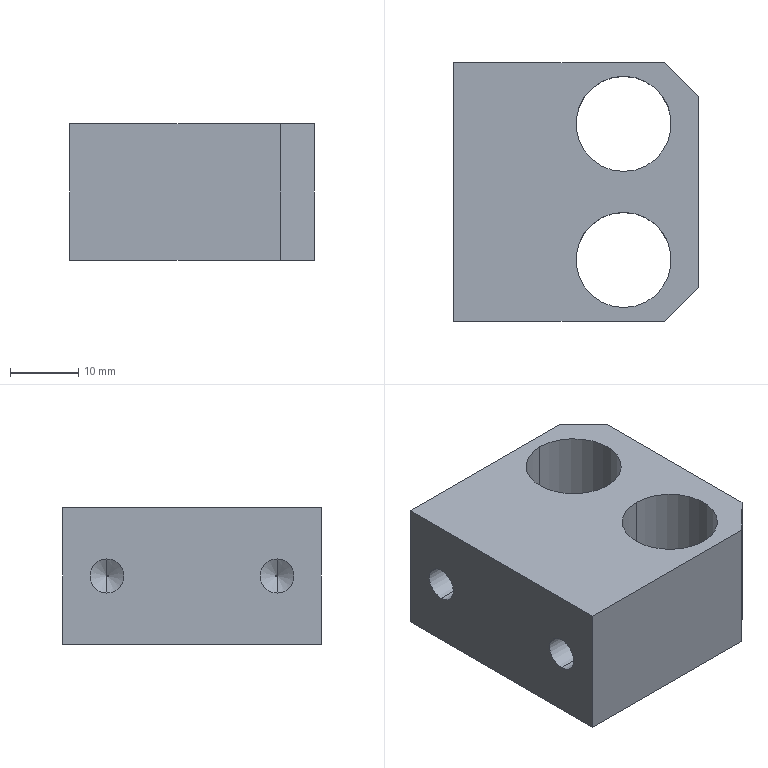Component | SolidWorks | 51-1 | 1 solid | 20 faces | box 36 x 38 x 20 mm | volume 20015 mm3 | cylinder 8 | plane 8 | cone 4 | commonest cylinder face diameters 14 x4 5 x4
build123d program:
from build123d import *

# Parameters (mm, degrees)
SKETCH1_W             = 38
SKETCH1_H             = 36
BOSS_EXTRUDE1_DEPTH   = 20
M6_TAPPED_HOLE1_D     = 5
M6_TAPPED_HOLE1_DEPTH = 17
M6_TAPPED_HOLE1_TIP   = 1.502
SKETCH4_R             = 7
CUT_EXTRUDE1_DEPTH    = 20
CHAMFER1_SIZE         = 5


with BuildPart() as part:
    # Sketch1 → Boss-Extrude1 (new body)
    with BuildSketch(Plane.XY):
        Rectangle(SKETCH1_W, SKETCH1_H)
    extrude(amount=BOSS_EXTRUDE1_DEPTH)

    # M6 Tapped Hole1
    with Locations(Plane(origin=(0, 18, 0), x_dir=(1, 0, 0), z_dir=(0, 1, 0))):
        with Locations((-12.5, -10), (12.5, -10)):
            Hole(M6_TAPPED_HOLE1_D / 2, depth=M6_TAPPED_HOLE1_DEPTH)
            with Locations((0, 0, -(M6_TAPPED_HOLE1_DEPTH + M6_TAPPED_HOLE1_TIP / 2))):  # 118° drill point
                Cone(0, M6_TAPPED_HOLE1_D / 2, M6_TAPPED_HOLE1_TIP, mode=Mode.SUBTRACT)

    # Sketch4 → Cut-Extrude1 (cut)
    with BuildSketch(Plane.XY.offset(20)):
        with Locations((-10, -7)):
            Circle(SKETCH4_R)
        with Locations((10, -7)):
            Circle(SKETCH4_R)
    extrude(amount=-CUT_EXTRUDE1_DEPTH, mode=Mode.SUBTRACT)

    # Chamfer1
    chamfer1_edges = [part.edges().sort_by_distance(p)[0] for p in [
        (19, -18, 10),
        (-19, -18, 10),
    ]]
    chamfer(chamfer1_edges, length=CHAMFER1_SIZE)


solid = part.part

# Placed as in the assembly
solid = solid.moved(Location((-7, -28, 376.398), (0, 0, 90)))
STEP:
#1=CARTESIAN_POINT('',(-0.,-0.9843,14.819));
#2=VERTEX_POINT('',#1);
#3=CARTESIAN_POINT('',(0.,-0.4331,14.819));
#4=VERTEX_POINT('',#3);
#5=CARTESIAN_POINT('',(-0.,-0.7087,14.819));
#6=DIRECTION('',(0.,0.,1.));
#7=DIRECTION('',(0.,1.,0.));
#8=AXIS2_PLACEMENT_3D('',#5,#6,#7);
#9=CIRCLE('',#8,0.2756);
#10=EDGE_CURVE('',#2,#4,#9,.T.);
#11=ORIENTED_EDGE('',*,*,#10,.F.);
#12=CARTESIAN_POINT('',(-0.,-0.9843,15.606));
#13=VERTEX_POINT('',#12);
#14=CARTESIAN_POINT('',(-0.,-0.9843,14.819));
#15=DIRECTION('',(0.,0.,1.));
#16=VECTOR('',#15,39.37);
#17=LINE('',#14,#16);
#18=EDGE_CURVE('',#2,#13,#17,.T.);
#19=ORIENTED_EDGE('',*,*,#18,.T.);
#20=CARTESIAN_POINT('',(0.,-0.4331,15.606));
#21=VERTEX_POINT('',#20);
#22=CARTESIAN_POINT('',(-0.,-0.7087,15.606));
#23=DIRECTION('',(0.,0.,1.));
#24=DIRECTION('',(0.,1.,0.));
#25=AXIS2_PLACEMENT_3D('',#22,#23,#24);
#26=CIRCLE('',#25,0.2756);
#27=EDGE_CURVE('',#13,#21,#26,.T.);
#28=ORIENTED_EDGE('',*,*,#27,.T.);
#29=CARTESIAN_POINT('',(0.,-0.4331,14.819));
#30=DIRECTION('',(0.,0.,1.));
#31=VECTOR('',#30,39.37);
#32=LINE('',#29,#31);
#33=EDGE_CURVE('',#4,#21,#32,.T.);
#34=ORIENTED_EDGE('',*,*,#33,.F.);
#35=EDGE_LOOP('',(#11,#19,#28,#34));
#36=FACE_OUTER_BOUND('',#35,.T.);
#37=CARTESIAN_POINT('',(-0.,-0.7087,14.819));
#38=DIRECTION('',(0.,0.,1.));
#39=DIRECTION('',(0.,1.,0.));
#40=AXIS2_PLACEMENT_3D('',#37,#38,#39);
#41=CYLINDRICAL_SURFACE('',#40,0.2756);
#42=ADVANCED_FACE('',(#36),#41,.F.);
#43=CARTESIAN_POINT('',(-0.,-1.772,14.819));
#44=VERTEX_POINT('',#43);
#45=CARTESIAN_POINT('',(-0.,-1.22,14.819));
#46=VERTEX_POINT('',#45);
#47=CARTESIAN_POINT('',(-0.,-1.496,14.819));
#48=DIRECTION('',(0.,0.,1.));
#49=DIRECTION('',(0.,1.,0.));
#50=AXIS2_PLACEMENT_3D('',#47,#48,#49);
#51=CIRCLE('',#50,0.2756);
#52=EDGE_CURVE('',#44,#46,#51,.T.);
#53=ORIENTED_EDGE('',*,*,#52,.F.);
#54=CARTESIAN_POINT('',(-0.,-1.772,15.606));
#55=VERTEX_POINT('',#54);
#56=CARTESIAN_POINT('',(-0.,-1.772,14.819));
#57=DIRECTION('',(0.,0.,1.));
#58=VECTOR('',#57,39.37);
#59=LINE('',#56,#58);
#60=EDGE_CURVE('',#44,#55,#59,.T.);
#61=ORIENTED_EDGE('',*,*,#60,.T.);
#62=CARTESIAN_POINT('',(-0.,-1.22,15.606));
#63=VERTEX_POINT('',#62);
#64=CARTESIAN_POINT('',(-0.,-1.496,15.606));
#65=DIRECTION('',(0.,0.,1.));
#66=DIRECTION('',(0.,1.,0.));
#67=AXIS2_PLACEMENT_3D('',#64,#65,#66);
#68=CIRCLE('',#67,0.2756);
#69=EDGE_CURVE('',#55,#63,#68,.T.);
#70=ORIENTED_EDGE('',*,*,#69,.T.);
#71=CARTESIAN_POINT('',(-0.,-1.22,14.819));
#72=DIRECTION('',(0.,0.,1.));
#73=VECTOR('',#72,39.37);
#74=LINE('',#71,#73);
#75=EDGE_CURVE('',#46,#63,#74,.T.);
#76=ORIENTED_EDGE('',*,*,#75,.F.);
#77=EDGE_LOOP('',(#53,#61,#70,#76));
#78=FACE_OUTER_BOUND('',#77,.T.);
#79=CARTESIAN_POINT('',(-0.,-1.496,14.819));
#80=DIRECTION('',(0.,0.,1.));
#81=DIRECTION('',(0.,1.,0.));
#82=AXIS2_PLACEMENT_3D('',#79,#80,#81);
#83=CYLINDRICAL_SURFACE('',#82,0.2756);
#84=ADVANCED_FACE('',(#78),#83,.F.);
#85=CARTESIAN_POINT('',(-0.315,-1.594,15.114));
#86=VERTEX_POINT('',#85);
#87=CARTESIAN_POINT('',(-0.315,-1.594,15.311));
#88=VERTEX_POINT('',#87);
#89=CARTESIAN_POINT('',(-0.315,-1.594,15.213));
#90=DIRECTION('',(-1.,0.,0.));
#91=DIRECTION('',(0.,0.,1.));
#92=AXIS2_PLACEMENT_3D('',#89,#90,#91);
#93=CIRCLE('',#92,0.09843);
#94=EDGE_CURVE('',#86,#88,#93,.T.);
#95=ORIENTED_EDGE('',*,*,#94,.F.);
#96=CARTESIAN_POINT('',(-0.9843,-1.594,15.114));
#97=VERTEX_POINT('',#96);
#98=CARTESIAN_POINT('',(-0.9843,-1.594,15.114));
#99=DIRECTION('',(-1.,0.,0.));
#100=VECTOR('',#99,39.37);
#101=LINE('',#98,#100);
#102=EDGE_CURVE('',#86,#97,#101,.T.);
#103=ORIENTED_EDGE('',*,*,#102,.T.);
#104=CARTESIAN_POINT('',(-0.9843,-1.594,15.311));
#105=VERTEX_POINT('',#104);
#106=CARTESIAN_POINT('',(-0.9843,-1.594,15.213));
#107=DIRECTION('',(-1.,0.,0.));
#108=DIRECTION('',(0.,0.,1.));
#109=AXIS2_PLACEMENT_3D('',#106,#107,#108);
#110=CIRCLE('',#109,0.09843);
#111=EDGE_CURVE('',#97,#105,#110,.T.);
#112=ORIENTED_EDGE('',*,*,#111,.T.);
#113=CARTESIAN_POINT('',(-0.9843,-1.594,15.311));
#114=DIRECTION('',(-1.,0.,0.));
#115=VECTOR('',#114,39.37);
#116=LINE('',#113,#115);
#117=EDGE_CURVE('',#88,#105,#116,.T.);
#118=ORIENTED_EDGE('',*,*,#117,.F.);
#119=EDGE_LOOP('',(#95,#103,#112,#118));
#120=FACE_OUTER_BOUND('',#119,.T.);
#121=CARTESIAN_POINT('',(-0.9843,-1.594,15.213));
#122=DIRECTION('',(-1.,0.,0.));
#123=DIRECTION('',(0.,0.,1.));
#124=AXIS2_PLACEMENT_3D('',#121,#122,#123);
#125=CYLINDRICAL_SURFACE('',#124,0.09843);
#126=ADVANCED_FACE('',(#120),#125,.F.);
#127=CARTESIAN_POINT('',(-0.2574,-1.594,15.215));
#128=VERTEX_POINT('',#127);
#129=CARTESIAN_POINT('',(-0.2574,-1.594,15.21));
#130=VERTEX_POINT('',#129);
#131=CARTESIAN_POINT('',(-0.2574,-1.594,15.215));
#132=CARTESIAN_POINT('',(-0.2574,-1.595,15.215));
#133=CARTESIAN_POINT('',(-0.2574,-1.595,15.215));
#134=CARTESIAN_POINT('',(-0.2573,-1.595,15.215));
#135=CARTESIAN_POINT('',(-0.2572,-1.595,15.215));
#136=CARTESIAN_POINT('',(-0.2571,-1.595,15.215));
#137=CARTESIAN_POINT('',(-0.257,-1.596,15.214));
#138=CARTESIAN_POINT('',(-0.2569,-1.596,15.214));
#139=CARTESIAN_POINT('',(-0.2569,-1.596,15.214));
#140=CARTESIAN_POINT('',(-0.2568,-1.596,15.213));
#141=CARTESIAN_POINT('',(-0.2568,-1.596,15.213));
#142=CARTESIAN_POINT('',(-0.2568,-1.596,15.213));
#143=CARTESIAN_POINT('',(-0.2568,-1.596,15.212));
#144=CARTESIAN_POINT('',(-0.2568,-1.596,15.212));
#145=CARTESIAN_POINT('',(-0.2568,-1.596,15.212));
#146=CARTESIAN_POINT('',(-0.2569,-1.596,15.212));
#147=CARTESIAN_POINT('',(-0.2569,-1.596,15.211));
#148=CARTESIAN_POINT('',(-0.257,-1.596,15.211));
#149=CARTESIAN_POINT('',(-0.257,-1.596,15.211));
#150=CARTESIAN_POINT('',(-0.2571,-1.595,15.21));
#151=CARTESIAN_POINT('',(-0.2572,-1.595,15.21));
#152=CARTESIAN_POINT('',(-0.2574,-1.595,15.21));
#153=CARTESIAN_POINT('',(-0.2574,-1.595,15.21));
#154=CARTESIAN_POINT('',(-0.2574,-1.595,15.21));
#155=CARTESIAN_POINT('',(-0.2574,-1.594,15.21));
#156=B_SPLINE_CURVE_WITH_KNOTS('',3,(#131,#132,#133,#134,#135,#136,#137,#138,#139,#140,#141,#142,#143,#144,#145,#146,#147,#148,#149,#150,#151,#152,#153,#154,#155),.UNSPECIFIED.,.F.,.F.,(4,3,3,3,3,3,3,3,4),(0.0004611,0.0004672,0.0004984,0.0005231,0.000548,0.0005696,0.0005914,0.0006239,0.0006283),.UNSPECIFIED.);
#157=EDGE_CURVE('',#128,#130,#156,.T.);
#158=ORIENTED_EDGE('',*,*,#157,.T.);
#159=CARTESIAN_POINT('',(-0.315,-1.594,15.114));
#160=DIRECTION('',(-0.515,0.,-0.8572));
#161=VECTOR('',#160,39.37);
#162=LINE('',#159,#161);
#163=EDGE_CURVE('',#130,#86,#162,.T.);
#164=ORIENTED_EDGE('',*,*,#163,.T.);
#165=ORIENTED_EDGE('',*,*,#94,.T.);
#166=CARTESIAN_POINT('',(-0.315,-1.594,15.311));
#167=DIRECTION('',(-0.515,0.,0.8572));
#168=VECTOR('',#167,39.37);
#169=LINE('',#166,#168);
#170=EDGE_CURVE('',#128,#88,#169,.T.);
#171=ORIENTED_EDGE('',*,*,#170,.F.);
#172=EDGE_LOOP('',(#158,#164,#165,#171));
#173=FACE_OUTER_BOUND('',#172,.T.);
#174=CARTESIAN_POINT('',(-0.315,-1.594,15.213));
#175=DIRECTION('',(-1.,0.,0.));
#176=DIRECTION('',(0.,0.,1.));
#177=AXIS2_PLACEMENT_3D('',#174,#175,#176);
#178=CONICAL_SURFACE('',#177,0.09843,1.03);
#179=ADVANCED_FACE('',(#173),#178,.F.);
#180=CARTESIAN_POINT('',(-0.315,-0.6102,15.114));
#181=VERTEX_POINT('',#180);
#182=CARTESIAN_POINT('',(-0.315,-0.6102,15.311));
#183=VERTEX_POINT('',#182);
#184=CARTESIAN_POINT('',(-0.315,-0.6102,15.213));
#185=DIRECTION('',(-1.,0.,0.));
#186=DIRECTION('',(0.,0.,1.));
#187=AXIS2_PLACEMENT_3D('',#184,#185,#186);
#188=CIRCLE('',#187,0.09843);
#189=EDGE_CURVE('',#181,#183,#188,.T.);
#190=ORIENTED_EDGE('',*,*,#189,.F.);
#191=CARTESIAN_POINT('',(-0.9843,-0.6102,15.114));
#192=VERTEX_POINT('',#191);
#193=CARTESIAN_POINT('',(-0.9843,-0.6102,15.114));
#194=DIRECTION('',(-1.,0.,0.));
#195=VECTOR('',#194,39.37);
#196=LINE('',#193,#195);
#197=EDGE_CURVE('',#181,#192,#196,.T.);
#198=ORIENTED_EDGE('',*,*,#197,.T.);
#199=CARTESIAN_POINT('',(-0.9843,-0.6102,15.311));
#200=VERTEX_POINT('',#199);
#201=CARTESIAN_POINT('',(-0.9843,-0.6102,15.213));
#202=DIRECTION('',(-1.,0.,0.));
#203=DIRECTION('',(0.,0.,1.));
#204=AXIS2_PLACEMENT_3D('',#201,#202,#203);
#205=CIRCLE('',#204,0.09843);
#206=EDGE_CURVE('',#192,#200,#205,.T.);
#207=ORIENTED_EDGE('',*,*,#206,.T.);
#208=CARTESIAN_POINT('',(-0.9843,-0.6102,15.311));
#209=DIRECTION('',(-1.,0.,0.));
#210=VECTOR('',#209,39.37);
#211=LINE('',#208,#210);
#212=EDGE_CURVE('',#183,#200,#211,.T.);
#213=ORIENTED_EDGE('',*,*,#212,.F.);
#214=EDGE_LOOP('',(#190,#198,#207,#213));
#215=FACE_OUTER_BOUND('',#214,.T.);
#216=CARTESIAN_POINT('',(-0.9843,-0.6102,15.213));
#217=DIRECTION('',(-1.,0.,0.));
#218=DIRECTION('',(0.,0.,1.));
#219=AXIS2_PLACEMENT_3D('',#216,#217,#218);
#220=CYLINDRICAL_SURFACE('',#219,0.09843);
#221=ADVANCED_FACE('',(#215),#220,.F.);
#222=CARTESIAN_POINT('',(-0.2574,-0.6102,15.215));
#223=VERTEX_POINT('',#222);
#224=CARTESIAN_POINT('',(-0.2574,-0.6102,15.21));
#225=VERTEX_POINT('',#224);
#226=CARTESIAN_POINT('',(-0.2574,-0.6102,15.215));
#227=CARTESIAN_POINT('',(-0.2576,-0.6106,15.215));
#228=CARTESIAN_POINT('',(-0.2577,-0.6111,15.216));
#229=CARTESIAN_POINT('',(-0.2579,-0.6116,15.216));
#230=CARTESIAN_POINT('',(-0.2581,-0.6121,15.216));
#231=CARTESIAN_POINT('',(-0.2583,-0.6126,15.216));
#232=CARTESIAN_POINT('',(-0.2585,-0.6132,15.216));
#233=CARTESIAN_POINT('',(-0.2587,-0.6138,15.216));
#234=CARTESIAN_POINT('',(-0.259,-0.6144,15.216));
#235=CARTESIAN_POINT('',(-0.2592,-0.615,15.215));
#236=CARTESIAN_POINT('',(-0.2593,-0.6154,15.215));
#237=CARTESIAN_POINT('',(-0.2595,-0.6158,15.215));
#238=CARTESIAN_POINT('',(-0.2596,-0.6161,15.215));
#239=CARTESIAN_POINT('',(-0.2597,-0.6163,15.214));
#240=CARTESIAN_POINT('',(-0.2597,-0.6166,15.214));
#241=CARTESIAN_POINT('',(-0.2598,-0.6167,15.214));
#242=CARTESIAN_POINT('',(-0.2599,-0.6169,15.214));
#243=CARTESIAN_POINT('',(-0.2599,-0.617,15.213));
#244=CARTESIAN_POINT('',(-0.2599,-0.617,15.213));
#245=CARTESIAN_POINT('',(-0.2599,-0.6171,15.213));
#246=CARTESIAN_POINT('',(-0.2599,-0.6171,15.212));
#247=CARTESIAN_POINT('',(-0.2599,-0.617,15.212));
#248=CARTESIAN_POINT('',(-0.2599,-0.617,15.212));
#249=CARTESIAN_POINT('',(-0.2598,-0.6168,15.211));
#250=CARTESIAN_POINT('',(-0.2598,-0.6167,15.211));
#251=CARTESIAN_POINT('',(-0.2597,-0.6165,15.211));
#252=CARTESIAN_POINT('',(-0.2596,-0.6163,15.21));
#253=CARTESIAN_POINT('',(-0.2596,-0.616,15.21));
#254=CARTESIAN_POINT('',(-0.2594,-0.6157,15.21));
#255=CARTESIAN_POINT('',(-0.2593,-0.6153,15.21));
#256=CARTESIAN_POINT('',(-0.2591,-0.6149,15.21));
#257=CARTESIAN_POINT('',(-0.2589,-0.6143,15.209));
#258=CARTESIAN_POINT('',(-0.2587,-0.6138,15.209));
#259=CARTESIAN_POINT('',(-0.2585,-0.6132,15.209));
#260=CARTESIAN_POINT('',(-0.2583,-0.6126,15.209));
#261=CARTESIAN_POINT('',(-0.2581,-0.612,15.209));
#262=CARTESIAN_POINT('',(-0.2579,-0.6115,15.209));
#263=CARTESIAN_POINT('',(-0.2577,-0.6111,15.209));
#264=CARTESIAN_POINT('',(-0.2576,-0.6106,15.21));
#265=CARTESIAN_POINT('',(-0.2574,-0.6102,15.21));
#266=B_SPLINE_CURVE_WITH_KNOTS('',3,(#226,#227,#228,#229,#230,#231,#232,#233,#234,#235,#236,#237,#238,#239,#240,#241,#242,#243,#244,#245,#246,#247,#248,#249,#250,#251,#252,#253,#254,#255,#256,#257,#258,#259,#260,#261,#262,#263,#264,#265),.UNSPECIFIED.,.F.,.F.,(4,3,3,3,3,3,3,3,3,3,3,3,3,4),(0.0003862,0.0004249,0.0004689,0.0005197,0.0005545,0.0005825,0.0006108,0.000631,0.0006576,0.0006838,0.0007204,0.0007665,0.0008131,0.00085),.UNSPECIFIED.);
#267=EDGE_CURVE('',#223,#225,#266,.T.);
#268=ORIENTED_EDGE('',*,*,#267,.T.);
#269=CARTESIAN_POINT('',(-0.315,-0.6102,15.114));
#270=DIRECTION('',(-0.515,0.,-0.8572));
#271=VECTOR('',#270,39.37);
#272=LINE('',#269,#271);
#273=EDGE_CURVE('',#225,#181,#272,.T.);
#274=ORIENTED_EDGE('',*,*,#273,.T.);
#275=ORIENTED_EDGE('',*,*,#189,.T.);
#276=CARTESIAN_POINT('',(-0.315,-0.6102,15.311));
#277=DIRECTION('',(-0.515,0.,0.8572));
#278=VECTOR('',#277,39.37);
#279=LINE('',#276,#278);
#280=EDGE_CURVE('',#223,#183,#279,.T.);
#281=ORIENTED_EDGE('',*,*,#280,.F.);
#282=EDGE_LOOP('',(#268,#274,#275,#281));
#283=FACE_OUTER_BOUND('',#282,.T.);
#284=CARTESIAN_POINT('',(-0.315,-0.6102,15.213));
#285=DIRECTION('',(-1.,0.,0.));
#286=DIRECTION('',(0.,0.,1.));
#287=AXIS2_PLACEMENT_3D('',#284,#285,#286);
#288=CONICAL_SURFACE('',#287,0.09843,1.03);
#289=ADVANCED_FACE('',(#283),#288,.F.);
#290=CARTESIAN_POINT('',(-0.9843,-1.85,14.819));
#291=VERTEX_POINT('',#290);
#292=CARTESIAN_POINT('',(0.2362,-1.85,14.819));
#293=VERTEX_POINT('',#292);
#294=CARTESIAN_POINT('',(-0.9843,-1.85,14.819));
#295=DIRECTION('',(1.,-0.,0.));
#296=VECTOR('',#295,39.37);
#297=LINE('',#294,#296);
#298=EDGE_CURVE('',#291,#293,#297,.T.);
#299=ORIENTED_EDGE('',*,*,#298,.T.);
#300=CARTESIAN_POINT('',(0.2362,-1.85,15.606));
#301=VERTEX_POINT('',#300);
#302=CARTESIAN_POINT('',(0.2362,-1.85,15.606));
#303=DIRECTION('',(0.,0.,1.));
#304=VECTOR('',#303,39.37);
#305=LINE('',#302,#304);
#306=EDGE_CURVE('',#293,#301,#305,.T.);
#307=ORIENTED_EDGE('',*,*,#306,.T.);
#308=CARTESIAN_POINT('',(-0.9843,-1.85,15.606));
#309=VERTEX_POINT('',#308);
#310=CARTESIAN_POINT('',(-0.9843,-1.85,15.606));
#311=DIRECTION('',(1.,-0.,0.));
#312=VECTOR('',#311,39.37);
#313=LINE('',#310,#312);
#314=EDGE_CURVE('',#309,#301,#313,.T.);
#315=ORIENTED_EDGE('',*,*,#314,.F.);
#316=CARTESIAN_POINT('',(-0.9843,-1.85,15.606));
#317=DIRECTION('',(0.,0.,-1.));
#318=VECTOR('',#317,39.37);
#319=LINE('',#316,#318);
#320=EDGE_CURVE('',#309,#291,#319,.T.);
#321=ORIENTED_EDGE('',*,*,#320,.T.);
#322=EDGE_LOOP('',(#299,#307,#315,#321));
#323=FACE_OUTER_BOUND('',#322,.T.);
#324=CARTESIAN_POINT('',(-0.9843,-1.85,15.606));
#325=DIRECTION('',(0.,1.,0.));
#326=DIRECTION('',(0.,0.,-1.));
#327=AXIS2_PLACEMENT_3D('',#324,#325,#326);
#328=PLANE('',#327);
#329=ADVANCED_FACE('',(#323),#328,.F.);
#330=CARTESIAN_POINT('',(0.4331,-1.654,15.606));
#331=VERTEX_POINT('',#330);
#332=CARTESIAN_POINT('',(0.4331,-0.5512,15.606));
#333=VERTEX_POINT('',#332);
#334=CARTESIAN_POINT('',(0.4331,-1.85,15.606));
#335=DIRECTION('',(0.,1.,0.));
#336=VECTOR('',#335,39.37);
#337=LINE('',#334,#336);
#338=EDGE_CURVE('',#331,#333,#337,.T.);
#339=ORIENTED_EDGE('',*,*,#338,.F.);
#340=CARTESIAN_POINT('',(0.4331,-1.654,14.819));
#341=VERTEX_POINT('',#340);
#342=CARTESIAN_POINT('',(0.4331,-1.654,15.606));
#343=DIRECTION('',(0.,0.,-1.));
#344=VECTOR('',#343,39.37);
#345=LINE('',#342,#344);
#346=EDGE_CURVE('',#331,#341,#345,.T.);
#347=ORIENTED_EDGE('',*,*,#346,.T.);
#348=CARTESIAN_POINT('',(0.4331,-0.5512,14.819));
#349=VERTEX_POINT('',#348);
#350=CARTESIAN_POINT('',(0.4331,-1.85,14.819));
#351=DIRECTION('',(0.,1.,0.));
#352=VECTOR('',#351,39.37);
#353=LINE('',#350,#352);
#354=EDGE_CURVE('',#341,#349,#353,.T.);
#355=ORIENTED_EDGE('',*,*,#354,.T.);
#356=CARTESIAN_POINT('',(0.4331,-0.5512,15.606));
#357=DIRECTION('',(0.,0.,1.));
#358=VECTOR('',#357,39.37);
#359=LINE('',#356,#358);
#360=EDGE_CURVE('',#349,#333,#359,.T.);
#361=ORIENTED_EDGE('',*,*,#360,.T.);
#362=EDGE_LOOP('',(#339,#347,#355,#361));
#363=FACE_OUTER_BOUND('',#362,.T.);
#364=CARTESIAN_POINT('',(0.4331,-1.85,15.606));
#365=DIRECTION('',(-1.,0.,0.));
#366=DIRECTION('',(0.,0.,1.));
#367=AXIS2_PLACEMENT_3D('',#364,#365,#366);
#368=PLANE('',#367);
#369=ADVANCED_FACE('',(#363),#368,.F.);
#370=CARTESIAN_POINT('',(0.2362,-0.3543,15.606));
#371=VERTEX_POINT('',#370);
#372=CARTESIAN_POINT('',(-0.9843,-0.3543,15.606));
#373=VERTEX_POINT('',#372);
#374=CARTESIAN_POINT('',(-0.9843,-0.3543,15.606));
#375=DIRECTION('',(-1.,0.,0.));
#376=VECTOR('',#375,39.37);
#377=LINE('',#374,#376);
#378=EDGE_CURVE('',#371,#373,#377,.T.);
#379=ORIENTED_EDGE('',*,*,#378,.F.);
#380=CARTESIAN_POINT('',(0.2362,-0.3543,14.819));
#381=VERTEX_POINT('',#380);
#382=CARTESIAN_POINT('',(0.2362,-0.3543,15.606));
#383=DIRECTION('',(0.,0.,-1.));
#384=VECTOR('',#383,39.37);
#385=LINE('',#382,#384);
#386=EDGE_CURVE('',#371,#381,#385,.T.);
#387=ORIENTED_EDGE('',*,*,#386,.T.);
#388=CARTESIAN_POINT('',(-0.9843,-0.3543,14.819));
#389=VERTEX_POINT('',#388);
#390=CARTESIAN_POINT('',(-0.9843,-0.3543,14.819));
#391=DIRECTION('',(-1.,0.,0.));
#392=VECTOR('',#391,39.37);
#393=LINE('',#390,#392);
#394=EDGE_CURVE('',#381,#389,#393,.T.);
#395=ORIENTED_EDGE('',*,*,#394,.T.);
#396=CARTESIAN_POINT('',(-0.9843,-0.3543,15.606));
#397=DIRECTION('',(0.,0.,-1.));
#398=VECTOR('',#397,39.37);
#399=LINE('',#396,#398);
#400=EDGE_CURVE('',#373,#389,#399,.T.);
#401=ORIENTED_EDGE('',*,*,#400,.F.);
#402=EDGE_LOOP('',(#379,#387,#395,#401));
#403=FACE_OUTER_BOUND('',#402,.T.);
#404=CARTESIAN_POINT('',(-0.9843,-0.3543,15.606));
#405=DIRECTION('',(-0.,-1.,0.));
#406=DIRECTION('',(1.,-0.,0.));
#407=AXIS2_PLACEMENT_3D('',#404,#405,#406);
#408=PLANE('',#407);
#409=ADVANCED_FACE('',(#403),#408,.F.);
#410=CARTESIAN_POINT('',(-0.9843,-1.594,15.213));
#411=DIRECTION('',(-1.,0.,0.));
#412=DIRECTION('',(0.,0.,1.));
#413=AXIS2_PLACEMENT_3D('',#410,#411,#412);
#414=CIRCLE('',#413,0.09843);
#415=EDGE_CURVE('',#105,#97,#414,.T.);
#416=ORIENTED_EDGE('',*,*,#415,.F.);
#417=ORIENTED_EDGE('',*,*,#111,.F.);
#418=EDGE_LOOP('',(#416,#417));
#419=FACE_BOUND('',#418,.T.);
#420=CARTESIAN_POINT('',(-0.9843,-0.6102,15.213));
#421=DIRECTION('',(-1.,0.,0.));
#422=DIRECTION('',(0.,0.,1.));
#423=AXIS2_PLACEMENT_3D('',#420,#421,#422);
#424=CIRCLE('',#423,0.09843);
#425=EDGE_CURVE('',#200,#192,#424,.T.);
#426=ORIENTED_EDGE('',*,*,#425,.F.);
#427=ORIENTED_EDGE('',*,*,#206,.F.);
#428=EDGE_LOOP('',(#426,#427));
#429=FACE_BOUND('',#428,.T.);
#430=CARTESIAN_POINT('',(-0.9843,-1.85,14.819));
#431=DIRECTION('',(-0.,-1.,0.));
#432=VECTOR('',#431,39.37);
#433=LINE('',#430,#432);
#434=EDGE_CURVE('',#389,#291,#433,.T.);
#435=ORIENTED_EDGE('',*,*,#434,.T.);
#436=ORIENTED_EDGE('',*,*,#320,.F.);
#437=CARTESIAN_POINT('',(-0.9843,-1.85,15.606));
#438=DIRECTION('',(-0.,-1.,0.));
#439=VECTOR('',#438,39.37);
#440=LINE('',#437,#439);
#441=EDGE_CURVE('',#373,#309,#440,.T.);
#442=ORIENTED_EDGE('',*,*,#441,.F.);
#443=ORIENTED_EDGE('',*,*,#400,.T.);
#444=EDGE_LOOP('',(#435,#436,#442,#443));
#445=FACE_OUTER_BOUND('',#444,.T.);
#446=CARTESIAN_POINT('',(-0.9843,-1.85,15.606));
#447=DIRECTION('',(1.,-0.,0.));
#448=DIRECTION('',(0.,0.,-1.));
#449=AXIS2_PLACEMENT_3D('',#446,#447,#448);
#450=PLANE('',#449);
#451=ADVANCED_FACE('',(#419,#429,#445),#450,.F.);
#452=CARTESIAN_POINT('',(-0.,-0.7087,15.606));
#453=DIRECTION('',(0.,0.,1.));
#454=DIRECTION('',(0.,1.,0.));
#455=AXIS2_PLACEMENT_3D('',#452,#453,#454);
#456=CIRCLE('',#455,0.2756);
#457=EDGE_CURVE('',#21,#13,#456,.T.);
#458=ORIENTED_EDGE('',*,*,#457,.F.);
#459=ORIENTED_EDGE('',*,*,#27,.F.);
#460=EDGE_LOOP('',(#458,#459));
#461=FACE_BOUND('',#460,.T.);
#462=CARTESIAN_POINT('',(-0.,-1.496,15.606));
#463=DIRECTION('',(0.,0.,1.));
#464=DIRECTION('',(0.,1.,0.));
#465=AXIS2_PLACEMENT_3D('',#462,#463,#464);
#466=CIRCLE('',#465,0.2756);
#467=EDGE_CURVE('',#63,#55,#466,.T.);
#468=ORIENTED_EDGE('',*,*,#467,.F.);
#469=ORIENTED_EDGE('',*,*,#69,.F.);
#470=EDGE_LOOP('',(#468,#469));
#471=FACE_BOUND('',#470,.T.);
#472=ORIENTED_EDGE('',*,*,#314,.T.);
#473=CARTESIAN_POINT('',(0.3543,-1.732,15.606));
#474=DIRECTION('',(0.7071,0.7071,0.));
#475=VECTOR('',#474,39.37);
#476=LINE('',#473,#475);
#477=EDGE_CURVE('',#301,#331,#476,.T.);
#478=ORIENTED_EDGE('',*,*,#477,.T.);
#479=ORIENTED_EDGE('',*,*,#338,.T.);
#480=CARTESIAN_POINT('',(0.3543,-0.4724,15.606));
#481=DIRECTION('',(-0.7071,0.7071,0.));
#482=VECTOR('',#481,39.37);
#483=LINE('',#480,#482);
#484=EDGE_CURVE('',#333,#371,#483,.T.);
#485=ORIENTED_EDGE('',*,*,#484,.T.);
#486=ORIENTED_EDGE('',*,*,#378,.T.);
#487=ORIENTED_EDGE('',*,*,#441,.T.);
#488=EDGE_LOOP('',(#472,#478,#479,#485,#486,#487));
#489=FACE_OUTER_BOUND('',#488,.T.);
#490=CARTESIAN_POINT('',(-0.2756,-1.102,15.606));
#491=DIRECTION('',(0.,0.,1.));
#492=DIRECTION('',(0.,1.,0.));
#493=AXIS2_PLACEMENT_3D('',#490,#491,#492);
#494=PLANE('',#493);
#495=ADVANCED_FACE('',(#461,#471,#489),#494,.T.);
#496=CARTESIAN_POINT('',(-0.,-0.7087,14.819));
#497=DIRECTION('',(0.,0.,1.));
#498=DIRECTION('',(0.,1.,0.));
#499=AXIS2_PLACEMENT_3D('',#496,#497,#498);
#500=CIRCLE('',#499,0.2756);
#501=EDGE_CURVE('',#4,#2,#500,.T.);
#502=ORIENTED_EDGE('',*,*,#501,.T.);
#503=ORIENTED_EDGE('',*,*,#10,.T.);
#504=EDGE_LOOP('',(#502,#503));
#505=FACE_BOUND('',#504,.T.);
#506=CARTESIAN_POINT('',(-0.,-1.496,14.819));
#507=DIRECTION('',(0.,0.,1.));
#508=DIRECTION('',(0.,1.,0.));
#509=AXIS2_PLACEMENT_3D('',#506,#507,#508);
#510=CIRCLE('',#509,0.2756);
#511=EDGE_CURVE('',#46,#44,#510,.T.);
#512=ORIENTED_EDGE('',*,*,#511,.T.);
#513=ORIENTED_EDGE('',*,*,#52,.T.);
#514=EDGE_LOOP('',(#512,#513));
#515=FACE_BOUND('',#514,.T.);
#516=ORIENTED_EDGE('',*,*,#354,.F.);
#517=CARTESIAN_POINT('',(0.4331,-1.654,14.819));
#518=DIRECTION('',(-0.7071,-0.7071,0.));
#519=VECTOR('',#518,39.37);
#520=LINE('',#517,#519);
#521=EDGE_CURVE('',#341,#293,#520,.T.);
#522=ORIENTED_EDGE('',*,*,#521,.T.);
#523=ORIENTED_EDGE('',*,*,#298,.F.);
#524=ORIENTED_EDGE('',*,*,#434,.F.);
#525=ORIENTED_EDGE('',*,*,#394,.F.);
#526=CARTESIAN_POINT('',(0.2362,-0.3543,14.819));
#527=DIRECTION('',(0.7071,-0.7071,0.));
#528=VECTOR('',#527,39.37);
#529=LINE('',#526,#528);
#530=EDGE_CURVE('',#381,#349,#529,.T.);
#531=ORIENTED_EDGE('',*,*,#530,.T.);
#532=EDGE_LOOP('',(#516,#522,#523,#524,#525,#531));
#533=FACE_OUTER_BOUND('',#532,.T.);
#534=CARTESIAN_POINT('',(-0.2756,-1.102,14.819));
#535=DIRECTION('',(0.,0.,1.));
#536=DIRECTION('',(0.,1.,0.));
#537=AXIS2_PLACEMENT_3D('',#534,#535,#536);
#538=PLANE('',#537);
#539=ADVANCED_FACE('',(#505,#515,#533),#538,.F.);
#540=ORIENTED_EDGE('',*,*,#273,.F.);
#541=CARTESIAN_POINT('',(-0.2574,-0.6102,15.21));
#542=CARTESIAN_POINT('',(-0.2574,-0.6102,15.21));
#543=CARTESIAN_POINT('',(-0.2574,-0.6101,15.21));
#544=CARTESIAN_POINT('',(-0.2573,-0.6101,15.21));
#545=CARTESIAN_POINT('',(-0.2572,-0.6097,15.21));
#546=CARTESIAN_POINT('',(-0.2571,-0.6094,15.211));
#547=CARTESIAN_POINT('',(-0.257,-0.6092,15.211));
#548=CARTESIAN_POINT('',(-0.2569,-0.609,15.211));
#549=CARTESIAN_POINT('',(-0.2569,-0.6089,15.211));
#550=CARTESIAN_POINT('',(-0.2568,-0.6088,15.212));
#551=CARTESIAN_POINT('',(-0.2568,-0.6087,15.212));
#552=CARTESIAN_POINT('',(-0.2568,-0.6086,15.212));
#553=CARTESIAN_POINT('',(-0.2568,-0.6086,15.213));
#554=CARTESIAN_POINT('',(-0.2568,-0.6086,15.213));
#555=CARTESIAN_POINT('',(-0.2568,-0.6087,15.213));
#556=CARTESIAN_POINT('',(-0.2569,-0.6088,15.213));
#557=CARTESIAN_POINT('',(-0.2569,-0.6089,15.214));
#558=CARTESIAN_POINT('',(-0.257,-0.609,15.214));
#559=CARTESIAN_POINT('',(-0.257,-0.6092,15.214));
#560=CARTESIAN_POINT('',(-0.2571,-0.6094,15.215));
#561=CARTESIAN_POINT('',(-0.2572,-0.6098,15.215));
#562=CARTESIAN_POINT('',(-0.2574,-0.6101,15.215));
#563=CARTESIAN_POINT('',(-0.2574,-0.6101,15.215));
#564=CARTESIAN_POINT('',(-0.2574,-0.6102,15.215));
#565=CARTESIAN_POINT('',(-0.2574,-0.6102,15.215));
#566=B_SPLINE_CURVE_WITH_KNOTS('',3,(#541,#542,#543,#544,#545,#546,#547,#548,#549,#550,#551,#552,#553,#554,#555,#556,#557,#558,#559,#560,#561,#562,#563,#564,#565),.UNSPECIFIED.,.F.,.F.,(4,3,3,3,3,3,3,3,4),(0.0002189,0.0002248,0.000256,0.0002808,0.0003057,0.0003274,0.0003492,0.0003816,0.0003862),.UNSPECIFIED.);
#567=EDGE_CURVE('',#225,#223,#566,.T.);
#568=ORIENTED_EDGE('',*,*,#567,.T.);
#569=ORIENTED_EDGE('',*,*,#280,.T.);
#570=CARTESIAN_POINT('',(-0.315,-0.6102,15.213));
#571=DIRECTION('',(-1.,0.,0.));
#572=DIRECTION('',(0.,0.,1.));
#573=AXIS2_PLACEMENT_3D('',#570,#571,#572);
#574=CIRCLE('',#573,0.09843);
#575=EDGE_CURVE('',#183,#181,#574,.T.);
#576=ORIENTED_EDGE('',*,*,#575,.T.);
#577=EDGE_LOOP('',(#540,#568,#569,#576));
#578=FACE_OUTER_BOUND('',#577,.T.);
#579=CARTESIAN_POINT('',(-0.315,-0.6102,15.213));
#580=DIRECTION('',(-1.,0.,0.));
#581=DIRECTION('',(0.,0.,1.));
#582=AXIS2_PLACEMENT_3D('',#579,#580,#581);
#583=CONICAL_SURFACE('',#582,0.09843,1.03);
#584=ADVANCED_FACE('',(#578),#583,.F.);
#585=ORIENTED_EDGE('',*,*,#197,.F.);
#586=ORIENTED_EDGE('',*,*,#575,.F.);
#587=ORIENTED_EDGE('',*,*,#212,.T.);
#588=ORIENTED_EDGE('',*,*,#425,.T.);
#589=EDGE_LOOP('',(#585,#586,#587,#588));
#590=FACE_OUTER_BOUND('',#589,.T.);
#591=CARTESIAN_POINT('',(-0.9843,-0.6102,15.213));
#592=DIRECTION('',(-1.,0.,0.));
#593=DIRECTION('',(0.,0.,1.));
#594=AXIS2_PLACEMENT_3D('',#591,#592,#593);
#595=CYLINDRICAL_SURFACE('',#594,0.09843);
#596=ADVANCED_FACE('',(#590),#595,.F.);
#597=ORIENTED_EDGE('',*,*,#163,.F.);
#598=CARTESIAN_POINT('',(-0.2574,-1.594,15.21));
#599=CARTESIAN_POINT('',(-0.2574,-1.594,15.21));
#600=CARTESIAN_POINT('',(-0.2574,-1.594,15.21));
#601=CARTESIAN_POINT('',(-0.2575,-1.594,15.21));
#602=CARTESIAN_POINT('',(-0.2576,-1.594,15.21));
#603=CARTESIAN_POINT('',(-0.2578,-1.594,15.209));
#604=CARTESIAN_POINT('',(-0.2579,-1.593,15.209));
#605=CARTESIAN_POINT('',(-0.2581,-1.593,15.209));
#606=CARTESIAN_POINT('',(-0.2584,-1.592,15.209));
#607=CARTESIAN_POINT('',(-0.2586,-1.591,15.209));
#608=CARTESIAN_POINT('',(-0.2588,-1.591,15.209));
#609=CARTESIAN_POINT('',(-0.259,-1.59,15.209));
#610=CARTESIAN_POINT('',(-0.2592,-1.59,15.21));
#611=CARTESIAN_POINT('',(-0.2594,-1.589,15.21));
#612=CARTESIAN_POINT('',(-0.2595,-1.589,15.21));
#613=CARTESIAN_POINT('',(-0.2596,-1.589,15.21));
#614=CARTESIAN_POINT('',(-0.2597,-1.588,15.211));
#615=CARTESIAN_POINT('',(-0.2598,-1.588,15.211));
#616=CARTESIAN_POINT('',(-0.2598,-1.588,15.211));
#617=CARTESIAN_POINT('',(-0.2599,-1.588,15.212));
#618=CARTESIAN_POINT('',(-0.2599,-1.588,15.212));
#619=CARTESIAN_POINT('',(-0.2599,-1.588,15.212));
#620=CARTESIAN_POINT('',(-0.2599,-1.588,15.213));
#621=CARTESIAN_POINT('',(-0.2599,-1.588,15.213));
#622=CARTESIAN_POINT('',(-0.2599,-1.588,15.213));
#623=CARTESIAN_POINT('',(-0.2599,-1.588,15.214));
#624=CARTESIAN_POINT('',(-0.2598,-1.588,15.214));
#625=CARTESIAN_POINT('',(-0.2598,-1.588,15.214));
#626=CARTESIAN_POINT('',(-0.2597,-1.588,15.214));
#627=CARTESIAN_POINT('',(-0.2596,-1.588,15.215));
#628=CARTESIAN_POINT('',(-0.2595,-1.589,15.215));
#629=CARTESIAN_POINT('',(-0.2594,-1.589,15.215));
#630=CARTESIAN_POINT('',(-0.2593,-1.589,15.215));
#631=CARTESIAN_POINT('',(-0.2591,-1.59,15.216));
#632=CARTESIAN_POINT('',(-0.2589,-1.59,15.216));
#633=CARTESIAN_POINT('',(-0.2587,-1.591,15.216));
#634=CARTESIAN_POINT('',(-0.2585,-1.592,15.216));
#635=CARTESIAN_POINT('',(-0.2583,-1.592,15.216));
#636=CARTESIAN_POINT('',(-0.2581,-1.593,15.216));
#637=CARTESIAN_POINT('',(-0.2579,-1.593,15.216));
#638=CARTESIAN_POINT('',(-0.2577,-1.594,15.216));
#639=CARTESIAN_POINT('',(-0.2576,-1.594,15.215));
#640=CARTESIAN_POINT('',(-0.2574,-1.594,15.215));
#641=B_SPLINE_CURVE_WITH_KNOTS('',3,(#598,#599,#600,#601,#602,#603,#604,#605,#606,#607,#608,#609,#610,#611,#612,#613,#614,#615,#616,#617,#618,#619,#620,#621,#622,#623,#624,#625,#626,#627,#628,#629,#630,#631,#632,#633,#634,#635,#636,#637,#638,#639,#640),.UNSPECIFIED.,.F.,.F.,(4,3,3,3,3,3,3,3,3,3,3,3,3,3,4),(0.0006283,0.0006313,0.0006688,0.0007142,0.0007651,0.0007993,0.0008269,0.0008548,0.0008787,0.0009015,0.0009264,0.000963,0.001009,0.001056,0.001092),.UNSPECIFIED.);
#642=EDGE_CURVE('',#130,#128,#641,.T.);
#643=ORIENTED_EDGE('',*,*,#642,.T.);
#644=ORIENTED_EDGE('',*,*,#170,.T.);
#645=CARTESIAN_POINT('',(-0.315,-1.594,15.213));
#646=DIRECTION('',(-1.,0.,0.));
#647=DIRECTION('',(0.,0.,1.));
#648=AXIS2_PLACEMENT_3D('',#645,#646,#647);
#649=CIRCLE('',#648,0.09843);
#650=EDGE_CURVE('',#88,#86,#649,.T.);
#651=ORIENTED_EDGE('',*,*,#650,.T.);
#652=EDGE_LOOP('',(#597,#643,#644,#651));
#653=FACE_OUTER_BOUND('',#652,.T.);
#654=CARTESIAN_POINT('',(-0.315,-1.594,15.213));
#655=DIRECTION('',(-1.,0.,0.));
#656=DIRECTION('',(0.,0.,1.));
#657=AXIS2_PLACEMENT_3D('',#654,#655,#656);
#658=CONICAL_SURFACE('',#657,0.09843,1.03);
#659=ADVANCED_FACE('',(#653),#658,.F.);
#660=ORIENTED_EDGE('',*,*,#102,.F.);
#661=ORIENTED_EDGE('',*,*,#650,.F.);
#662=ORIENTED_EDGE('',*,*,#117,.T.);
#663=ORIENTED_EDGE('',*,*,#415,.T.);
#664=EDGE_LOOP('',(#660,#661,#662,#663));
#665=FACE_OUTER_BOUND('',#664,.T.);
#666=CARTESIAN_POINT('',(-0.9843,-1.594,15.213));
#667=DIRECTION('',(-1.,0.,0.));
#668=DIRECTION('',(0.,0.,1.));
#669=AXIS2_PLACEMENT_3D('',#666,#667,#668);
#670=CYLINDRICAL_SURFACE('',#669,0.09843);
#671=ADVANCED_FACE('',(#665),#670,.F.);
#672=ORIENTED_EDGE('',*,*,#60,.F.);
#673=ORIENTED_EDGE('',*,*,#511,.F.);
#674=ORIENTED_EDGE('',*,*,#75,.T.);
#675=ORIENTED_EDGE('',*,*,#467,.T.);
#676=EDGE_LOOP('',(#672,#673,#674,#675));
#677=FACE_OUTER_BOUND('',#676,.T.);
#678=ORIENTED_EDGE('',*,*,#157,.F.);
#679=ORIENTED_EDGE('',*,*,#642,.F.);
#680=EDGE_LOOP('',(#678,#679));
#681=FACE_BOUND('',#680,.T.);
#682=CARTESIAN_POINT('',(-0.,-1.496,14.819));
#683=DIRECTION('',(0.,0.,1.));
#684=DIRECTION('',(0.,1.,0.));
#685=AXIS2_PLACEMENT_3D('',#682,#683,#684);
#686=CYLINDRICAL_SURFACE('',#685,0.2756);
#687=ADVANCED_FACE('',(#677,#681),#686,.F.);
#688=ORIENTED_EDGE('',*,*,#18,.F.);
#689=ORIENTED_EDGE('',*,*,#501,.F.);
#690=ORIENTED_EDGE('',*,*,#33,.T.);
#691=ORIENTED_EDGE('',*,*,#457,.T.);
#692=EDGE_LOOP('',(#688,#689,#690,#691));
#693=FACE_OUTER_BOUND('',#692,.T.);
#694=ORIENTED_EDGE('',*,*,#267,.F.);
#695=ORIENTED_EDGE('',*,*,#567,.F.);
#696=EDGE_LOOP('',(#694,#695));
#697=FACE_BOUND('',#696,.T.);
#698=CARTESIAN_POINT('',(-0.,-0.7087,14.819));
#699=DIRECTION('',(0.,0.,1.));
#700=DIRECTION('',(0.,1.,0.));
#701=AXIS2_PLACEMENT_3D('',#698,#699,#700);
#702=CYLINDRICAL_SURFACE('',#701,0.2756);
#703=ADVANCED_FACE('',(#693,#697),#702,.F.);
#704=ORIENTED_EDGE('',*,*,#477,.F.);
#705=ORIENTED_EDGE('',*,*,#306,.F.);
#706=ORIENTED_EDGE('',*,*,#521,.F.);
#707=ORIENTED_EDGE('',*,*,#346,.F.);
#708=EDGE_LOOP('',(#704,#705,#706,#707));
#709=FACE_OUTER_BOUND('',#708,.T.);
#710=CARTESIAN_POINT('',(0.4331,-1.654,15.606));
#711=DIRECTION('',(-0.7071,0.7071,0.));
#712=DIRECTION('',(0.,0.,-1.));
#713=AXIS2_PLACEMENT_3D('',#710,#711,#712);
#714=PLANE('',#713);
#715=ADVANCED_FACE('',(#709),#714,.F.);
#716=ORIENTED_EDGE('',*,*,#484,.F.);
#717=ORIENTED_EDGE('',*,*,#360,.F.);
#718=ORIENTED_EDGE('',*,*,#530,.F.);
#719=ORIENTED_EDGE('',*,*,#386,.F.);
#720=EDGE_LOOP('',(#716,#717,#718,#719));
#721=FACE_OUTER_BOUND('',#720,.T.);
#722=CARTESIAN_POINT('',(0.2362,-0.3543,15.606));
#723=DIRECTION('',(-0.7071,-0.7071,0.));
#724=DIRECTION('',(0.,0.,-1.));
#725=AXIS2_PLACEMENT_3D('',#722,#723,#724);
#726=PLANE('',#725);
#727=ADVANCED_FACE('',(#721),#726,.F.);
#728=CLOSED_SHELL('',(#42,#84,#126,#179,#221,#289,#329,#369,#409,#451,#495,#539,#584,#596,#659,#671,#687,#703,#715,#727));
#729=MANIFOLD_SOLID_BREP('',#728);
#730=CARTESIAN_POINT('',(0.,0.,0.));
#731=DIRECTION('',(0.,0.,1.));
#732=DIRECTION('',(1.,0.,0.));
#733=AXIS2_PLACEMENT_3D('',#730,#731,#732);
#734=(LENGTH_UNIT()NAMED_UNIT(*)SI_UNIT($,.METRE.));
#735=LENGTH_MEASURE_WITH_UNIT(LENGTH_MEASURE(0.0254),#734);
#736=DIMENSIONAL_EXPONENTS(1.,0.,0.,0.,0.,0.,0.);
#737=(CONVERSION_BASED_UNIT('',#735)LENGTH_UNIT()NAMED_UNIT(#736));
#738=UNCERTAINTY_MEASURE_WITH_UNIT(LENGTH_MEASURE(0.00001),#737,'','');
#739=(NAMED_UNIT(*)PLANE_ANGLE_UNIT()SI_UNIT($,.RADIAN.));
#740=(NAMED_UNIT(*)SI_UNIT($,.STERADIAN.)SOLID_ANGLE_UNIT());
#741=(GEOMETRIC_REPRESENTATION_CONTEXT(3)GLOBAL_UNCERTAINTY_ASSIGNED_CONTEXT((#738))GLOBAL_UNIT_ASSIGNED_CONTEXT((#737,#739,#740))REPRESENTATION_CONTEXT('',''));
#742=ADVANCED_BREP_SHAPE_REPRESENTATION('',(#729,#733),#741);
#743=COLOUR_RGB('',0.7922,0.8196,0.9333);
#744=FILL_AREA_STYLE_COLOUR('',#743);
#745=FILL_AREA_STYLE('',(#744));
#746=SURFACE_STYLE_FILL_AREA(#745);
#747=SURFACE_SIDE_STYLE('',(#746));
#748=SURFACE_STYLE_USAGE(.BOTH.,#747);
#749=PRESENTATION_STYLE_ASSIGNMENT((#748));
#750=STYLED_ITEM('',(#749),#729);
#751=(LENGTH_UNIT()NAMED_UNIT(*)SI_UNIT($,.METRE.));
#752=LENGTH_MEASURE_WITH_UNIT(LENGTH_MEASURE(0.0254),#751);
#753=DIMENSIONAL_EXPONENTS(1.,0.,0.,0.,0.,0.,0.);
#754=(CONVERSION_BASED_UNIT('',#752)LENGTH_UNIT()NAMED_UNIT(#753));
#755=UNCERTAINTY_MEASURE_WITH_UNIT(LENGTH_MEASURE(0.00001),#754,'','');
#756=(NAMED_UNIT(*)PLANE_ANGLE_UNIT()SI_UNIT($,.RADIAN.));
#757=(NAMED_UNIT(*)SI_UNIT($,.STERADIAN.)SOLID_ANGLE_UNIT());
#758=(GEOMETRIC_REPRESENTATION_CONTEXT(3)GLOBAL_UNCERTAINTY_ASSIGNED_CONTEXT((#755))GLOBAL_UNIT_ASSIGNED_CONTEXT((#754,#756,#757))REPRESENTATION_CONTEXT('',''));
#759=MECHANICAL_DESIGN_GEOMETRIC_PRESENTATION_REPRESENTATION('',(#750),#758);
#760=PRESENTATION_LAYER_ASSIGNMENT('','',(#750));